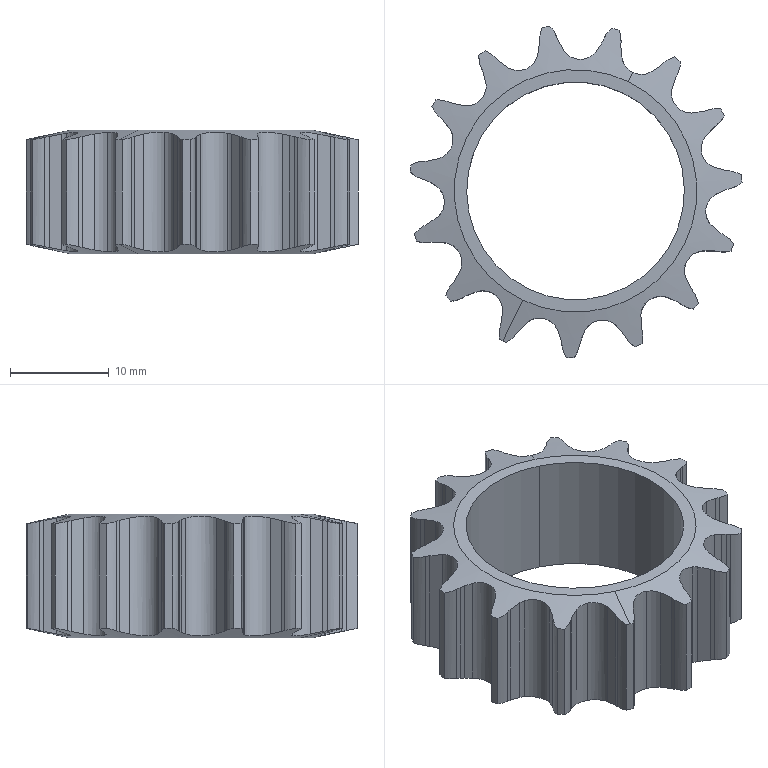Component | SolidWorks | Gear-DragChain-1 | 1 solid | 136 faces | volume 3543 mm3 | cylinder 100 | plane 32 | cone 4 | commonest cylinder face diameters 10.36 x32 6.643 x32 4.02 x19 33.684 x15 22 x2